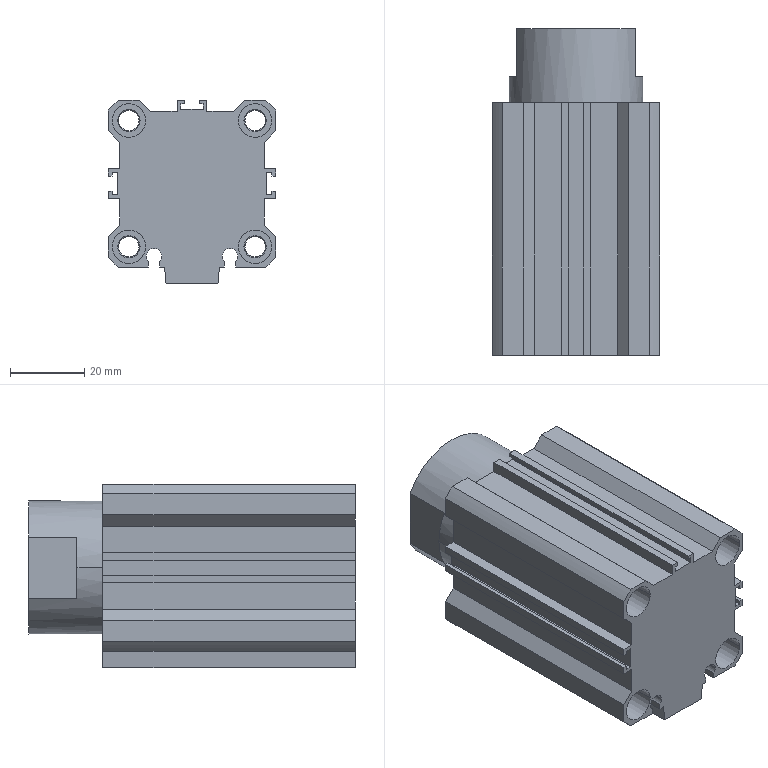Component | SolidWorks | RSDQA32-20DD-M9BL(0_0)-1_RSQA32-20D(0)_BODY-1 | 1 solid | 147 faces | volume 101302 mm3 | plane 79 | cylinder 44 | cone 24 | commonest cylinder face diameters 9 x16 5.5 x8 4.15 x6 8.566 x4 60 x4 36 x2 20 x2 32 x2